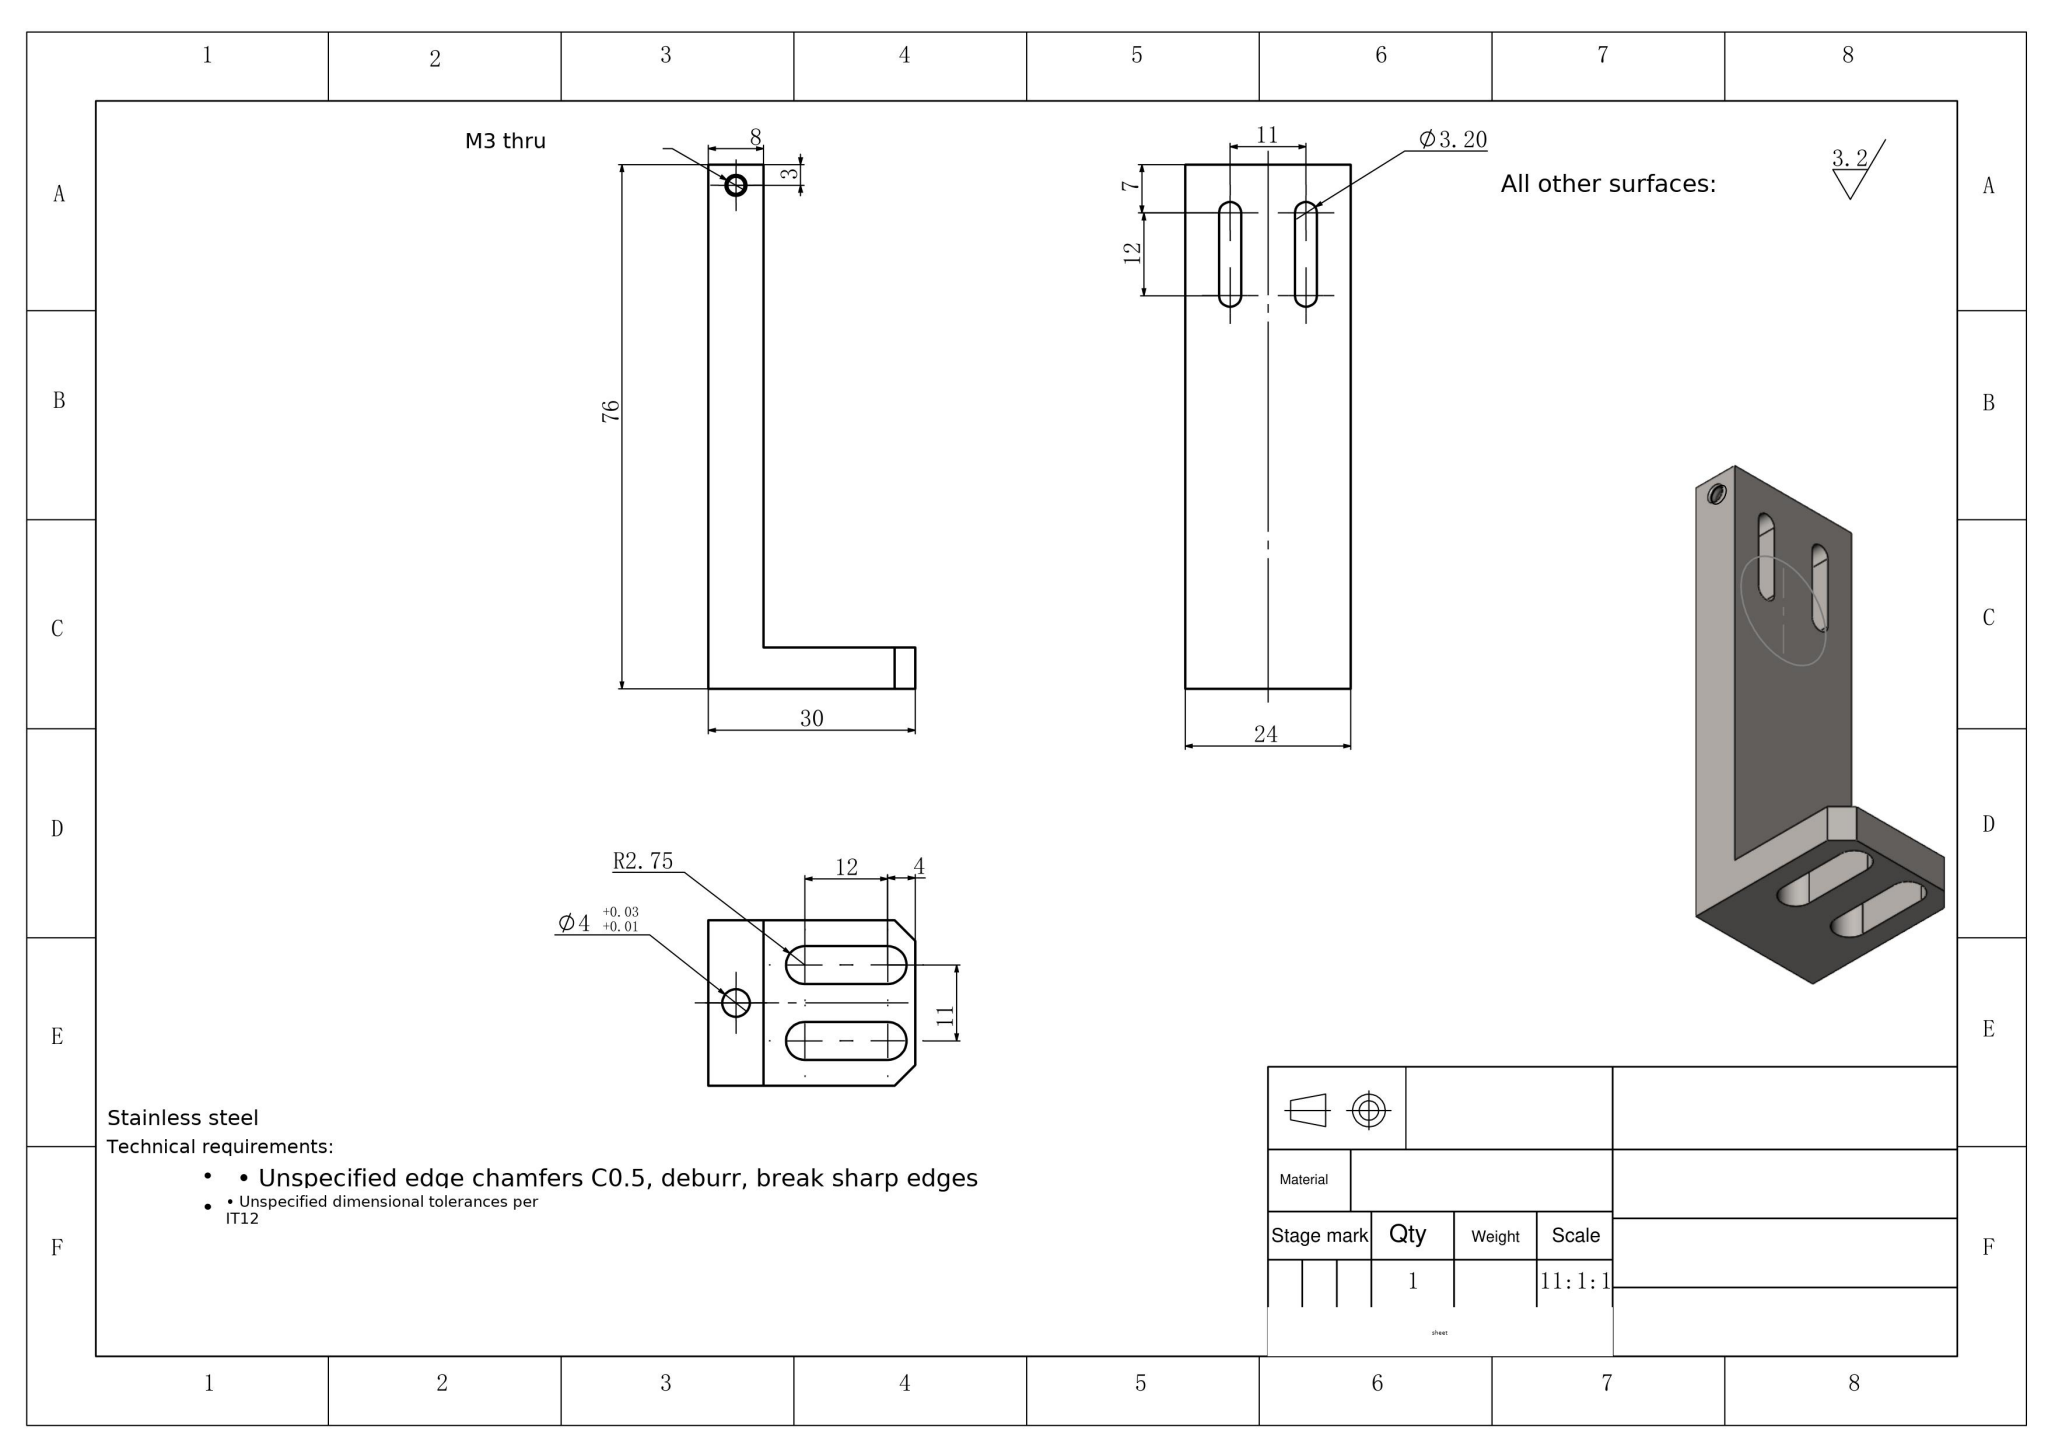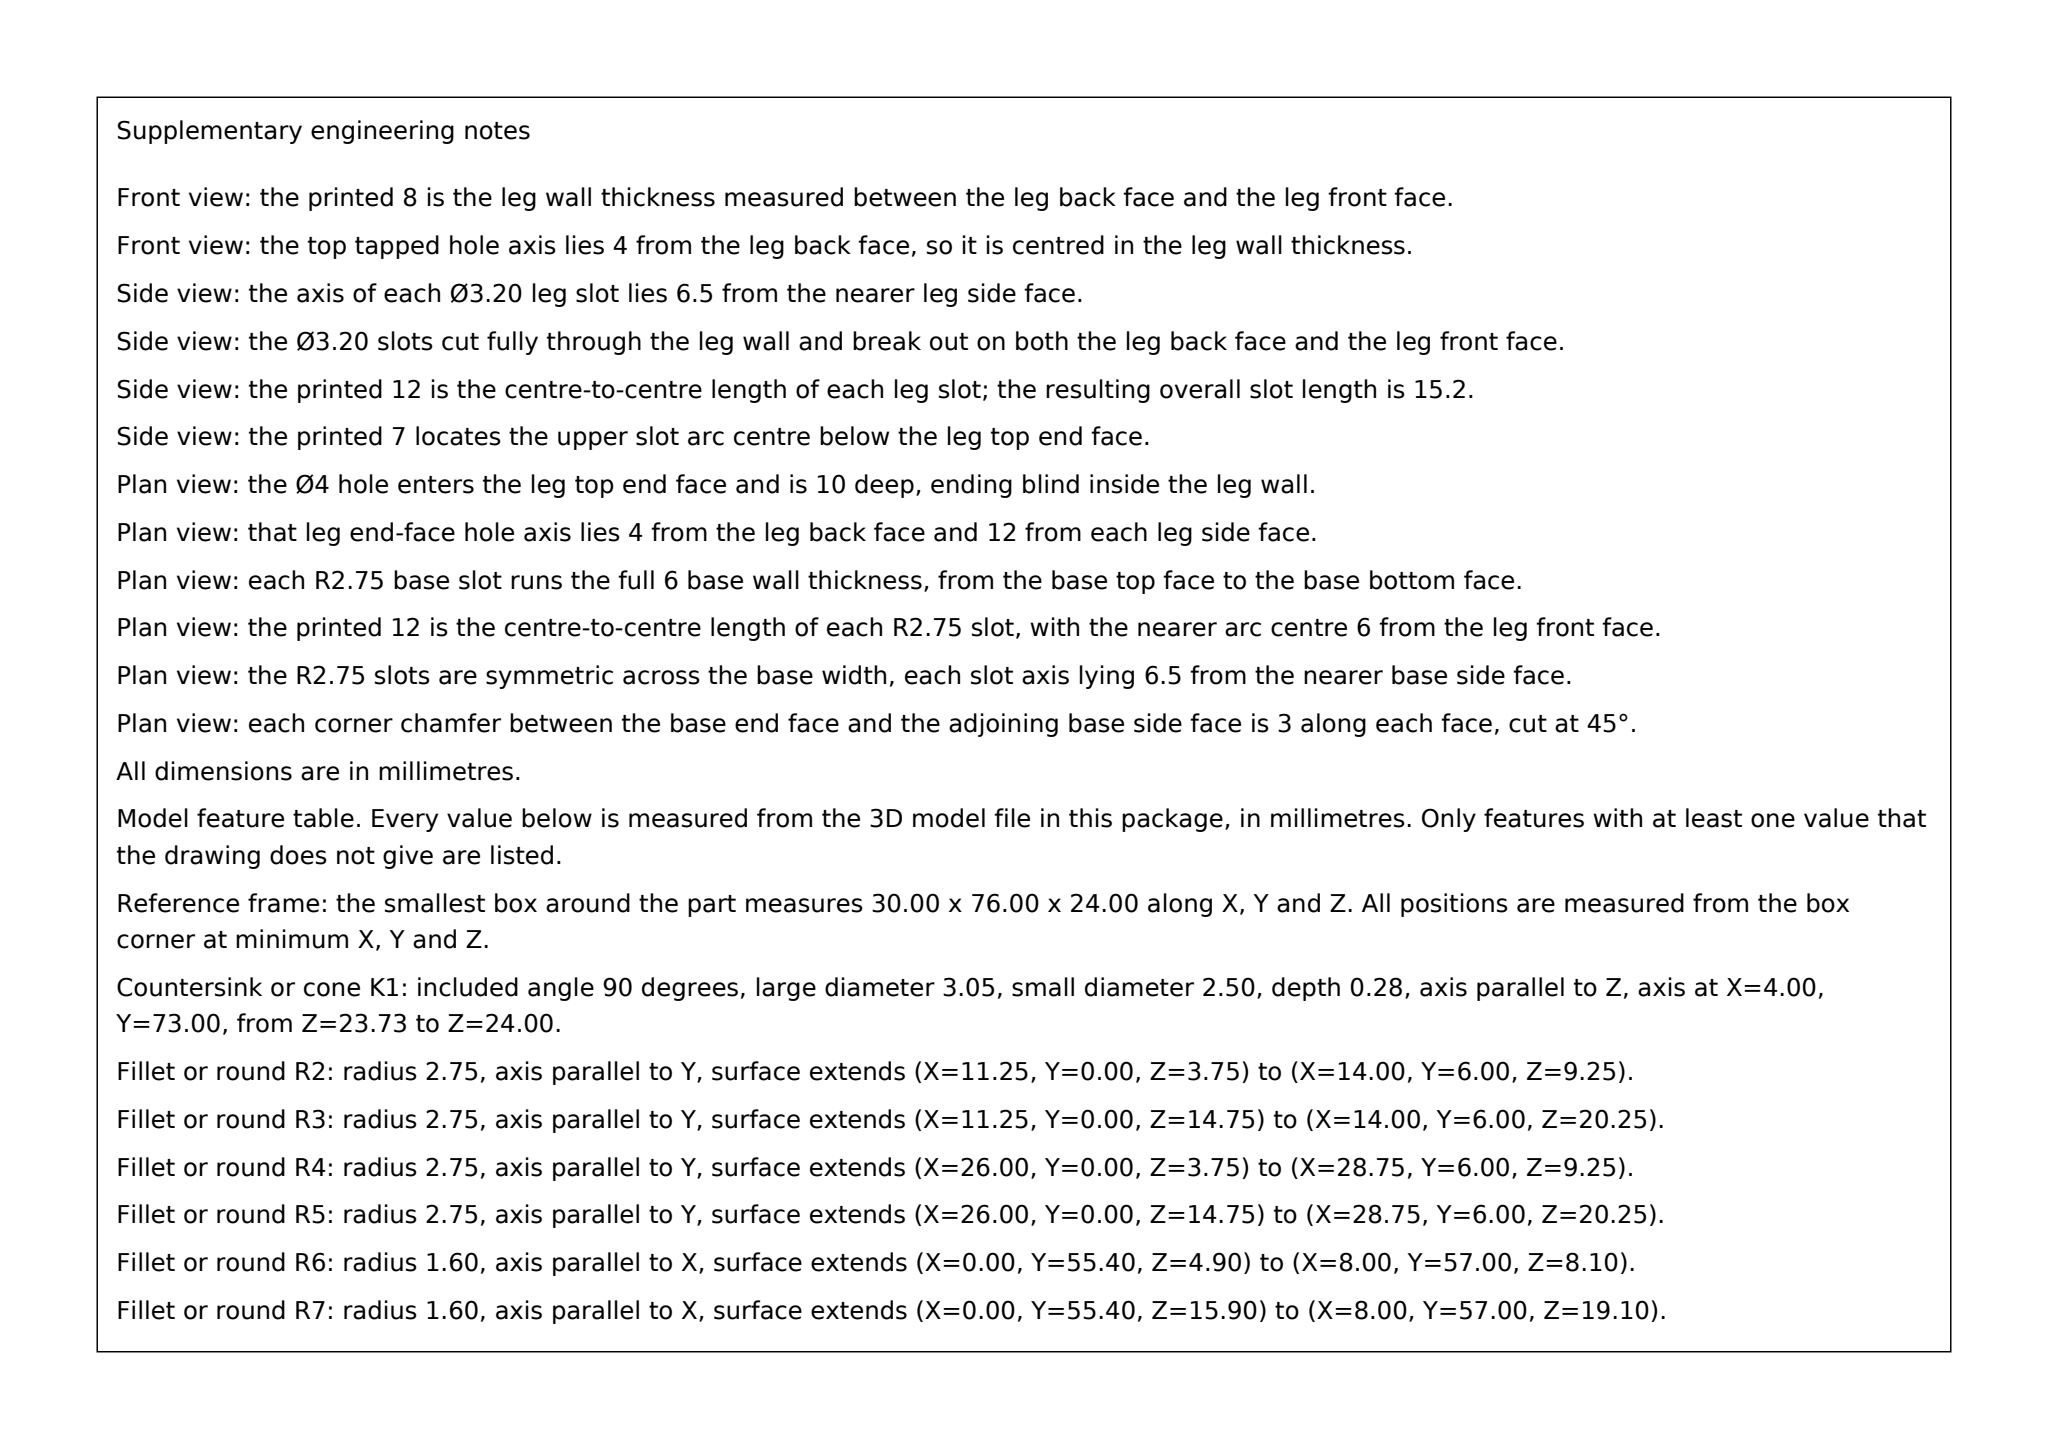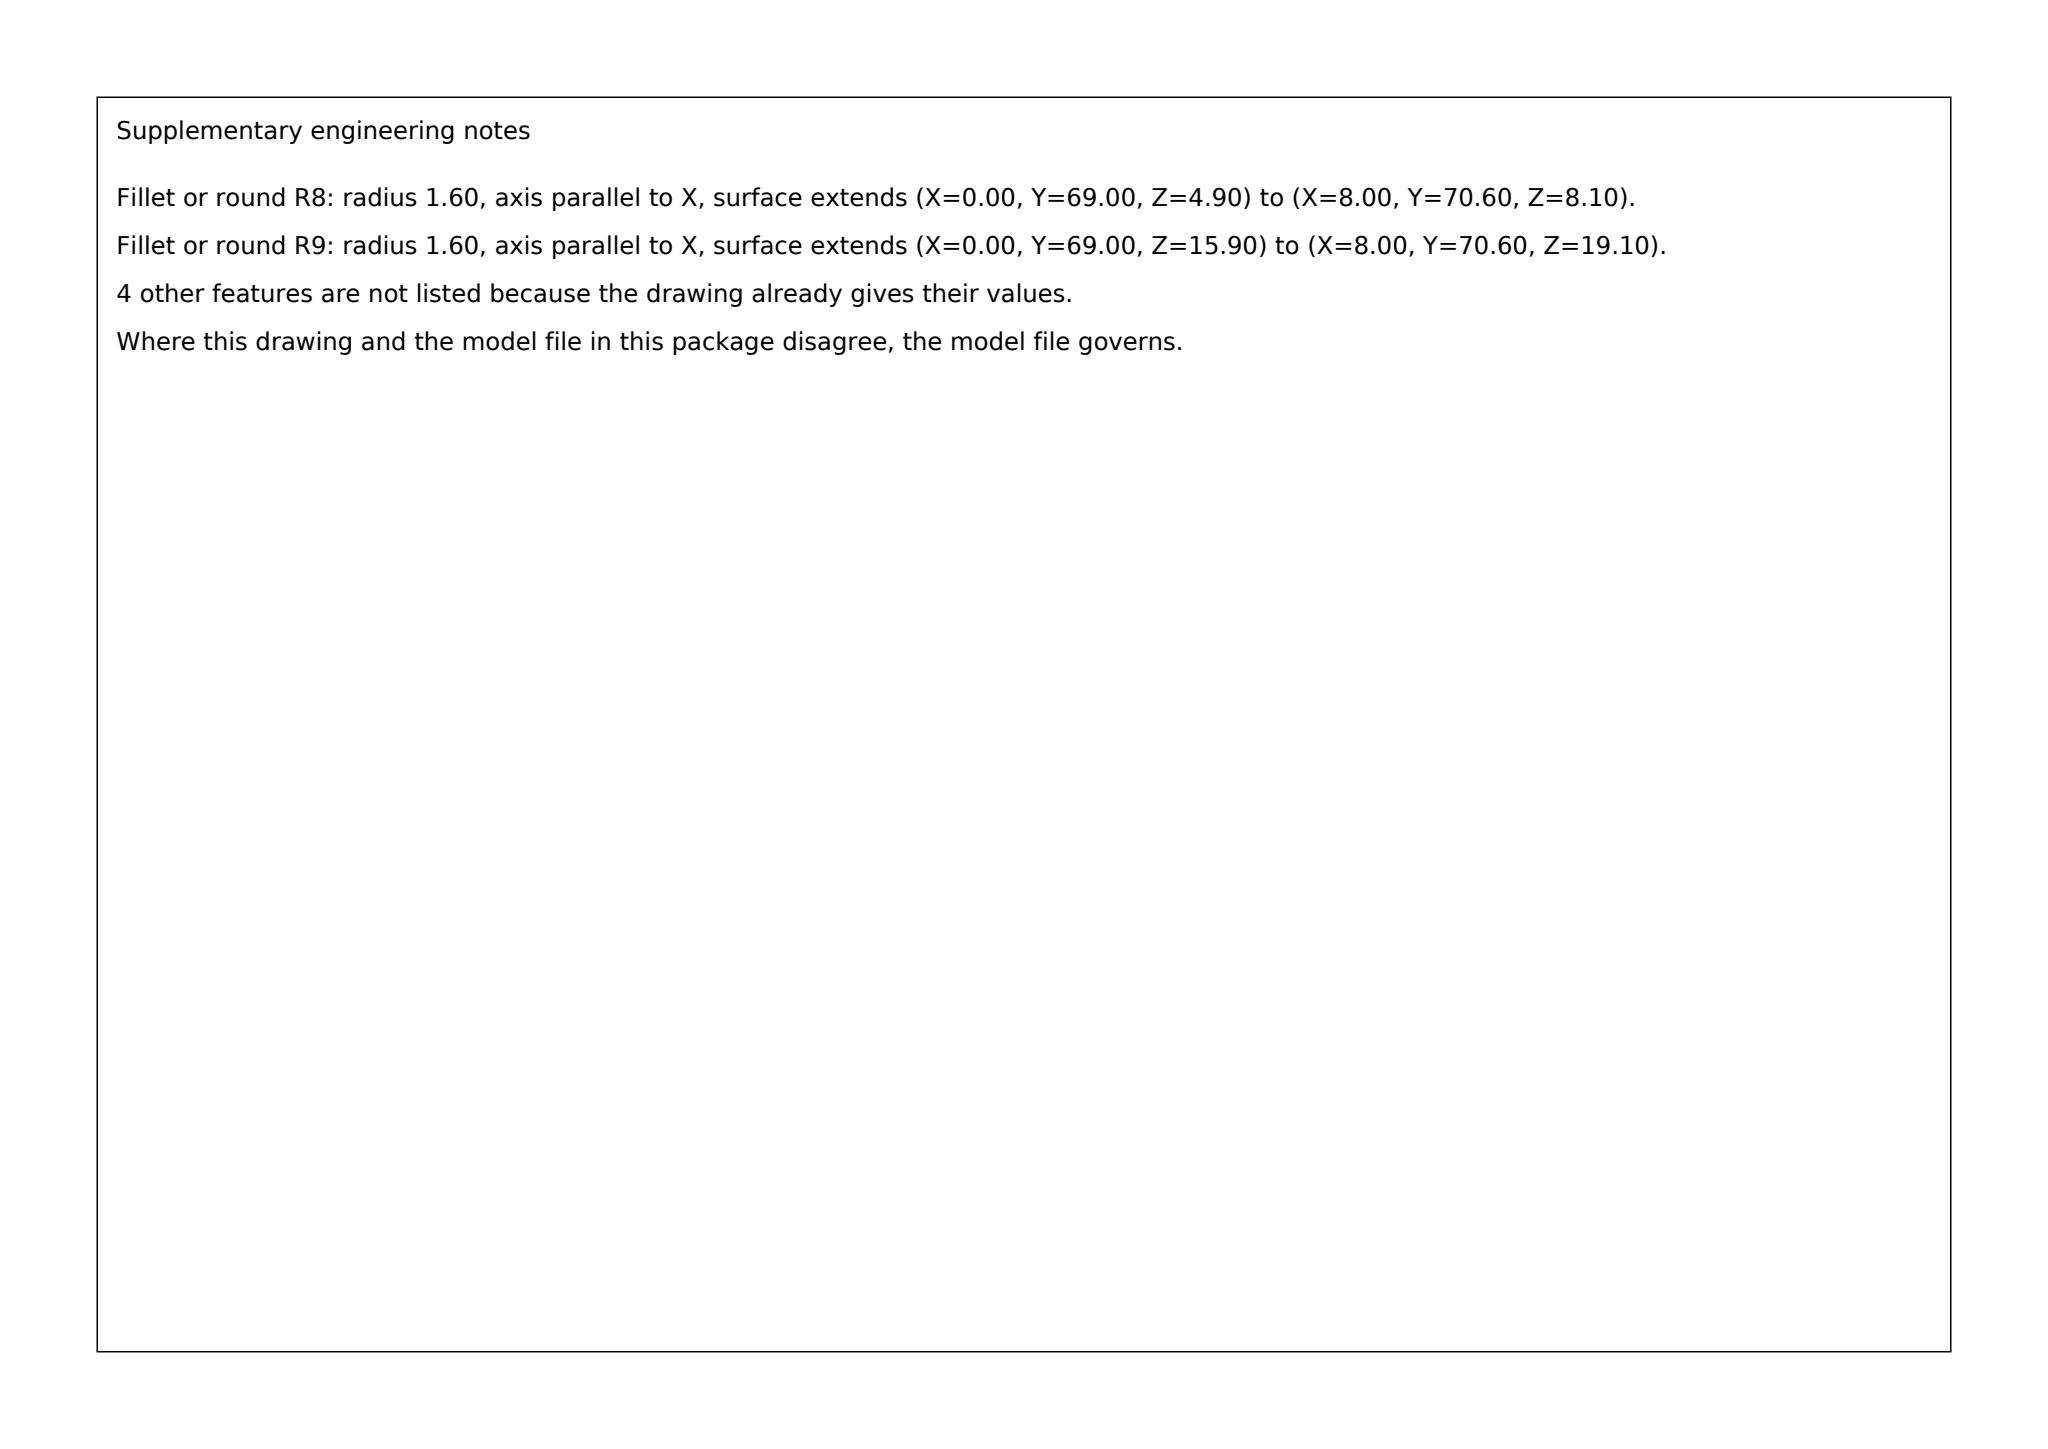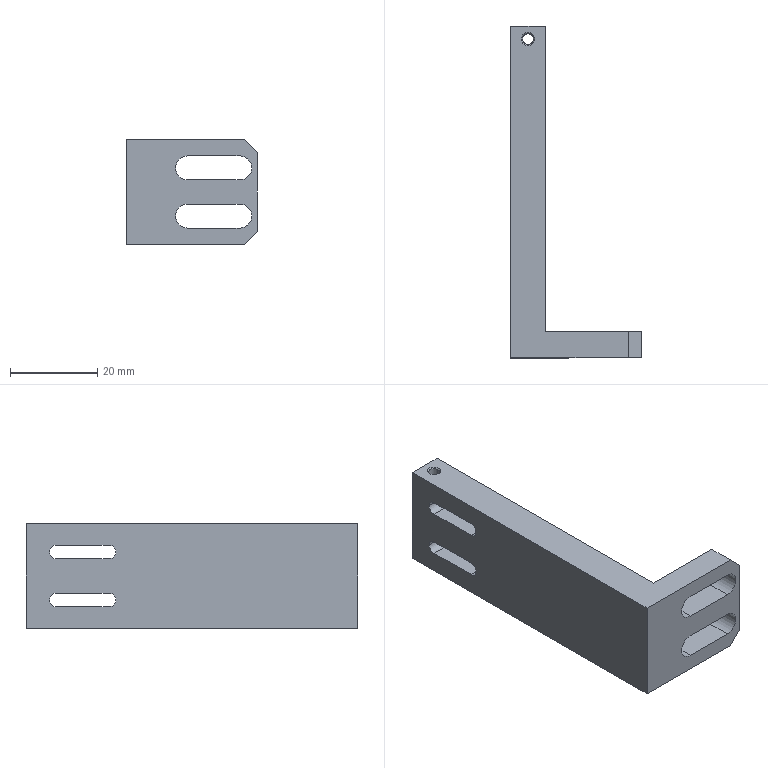Part | SolidWorks | mm | 1 solid | 39 faces | box 30 x 76 x 24 mm | volume 15661 mm3 | plane 19 | cylinder 18 | cone 2 | commonest cylinder face diameters 5.5 x6 3.2 x6 2.5 x4 4 x2
Drawing notes:
Ø4 +0.03/+0.01 hole in base: 10 deep (no counterbore), axis normal to base, located 4 from back face and 12 from either side face (centred in 24 width). | from the solid: cylinders[dia,axis,pos_other_axes,length]: [4.0,"y",[4.0,null,12.0],10.0]
M3 THRU: hole axis 4 from back face, i.e. centred in the 8 thick upright wall, and 3 from top face. | from the solid: cylinders[dia,axis,pos_other_axes,length]: [2.5,"z",[4.0,73.0,null],10.16/10.44] with planes x=0 and x=8
Base plate thickness 6 (from bottom face datum y=0 to underside of upright flange). | from the solid: axis_planes[normal_axis,offset]: y 0.0 and y 6.0
build123d program:
from build123d import *

# Parameters (mm, degrees)
BOSS_EXTRUDE1_DEPTH         = 24
CUT_EXTRUDE1_DEPTH          = 78.201
M3_TAPPED_HOLE1_D           = 2.5
M3_TAPPED_HOLE1_CSINK_D     = 3.05
M3_TAPPED_HOLE1_CSINK_ANGLE = 90
SKETCH5_R                   = 2
CUT_EXTRUDE2_DEPTH          = 10
CUT_EXTRUDE3_DEPTH          = 78.201
CHAMFER1_SIZE               = 3


with BuildPart() as part:
    # Sketch1 → Boss-Extrude1 (new body)
    with BuildSketch(Plane.XY):
        Polygon((0, 0), (0, 70), (-8, 70), (-8, -6), (22, -6), (22, 0), align=None)
    extrude(amount=BOSS_EXTRUDE1_DEPTH)

    # Sketch2 → Cut-Extrude1 (cut, through all)
    with BuildSketch(Plane(origin=(0, 0, 0), x_dir=(0, 0, -1), z_dir=(1, 0, 0))):
        with BuildLine():
            Line((-15.9, 63), (-15.9, 51))
            ThreePointArc((-15.9, 51), (-17.5, 49.4), (-19.1, 51))
            Line((-19.1, 51), (-19.1, 63))
            ThreePointArc((-19.1, 63), (-17.5, 64.6), (-15.9, 63))
        make_face()
        with BuildLine():
            Line((-4.9, 63), (-4.9, 51))
            ThreePointArc((-4.9, 51), (-6.5, 49.4), (-8.1, 51))
            Line((-8.1, 51), (-8.1, 63))
            ThreePointArc((-8.1, 63), (-6.5, 64.6), (-4.9, 63))
        make_face()
    extrude(amount=-CUT_EXTRUDE1_DEPTH, mode=Mode.SUBTRACT)

    # M3 Tapped Hole1 (through all)
    with Locations(Plane.XY.offset(24)):
        with Locations((-4, 67)):
            CounterSinkHole(M3_TAPPED_HOLE1_D / 2, M3_TAPPED_HOLE1_CSINK_D / 2, counter_sink_angle=M3_TAPPED_HOLE1_CSINK_ANGLE)

    # Sketch5 → Cut-Extrude2 (cut)
    with BuildSketch(Plane(origin=(0, 70, 0), x_dir=(1, 0, 0), z_dir=(0, 1, 0))):
        with Locations(Location((-4, -12, 0), (0, 0, 270))):
            Circle(SKETCH5_R)
    extrude(amount=-CUT_EXTRUDE2_DEPTH, mode=Mode.SUBTRACT)

    # Sketch6 → Cut-Extrude3 (cut, through all)
    with BuildSketch(Plane(origin=(0, 0, 0), x_dir=(1, 0, 0), z_dir=(0, 1, 0))):
        with BuildLine():
            Line((6, -14.75), (18, -14.75))
            ThreePointArc((18, -14.75), (20.75, -17.5), (18, -20.25))
            Line((18, -20.25), (6, -20.25))
            ThreePointArc((6, -20.25), (3.25, -17.5), (6, -14.75))
        make_face()
        with BuildLine():
            Line((6, -9.25), (18, -9.25))
            ThreePointArc((18, -9.25), (20.75, -6.5), (18, -3.75))
            Line((18, -3.75), (6, -3.75))
            ThreePointArc((6, -3.75), (3.25, -6.5), (6, -9.25))
        make_face()
    extrude(amount=-CUT_EXTRUDE3_DEPTH, mode=Mode.SUBTRACT)

    # Chamfer1
    chamfer1_edges = [part.edges().sort_by_distance(p)[0] for p in [
        (22, -3, 24),
        (22, -3, 0),
    ]]
    chamfer(chamfer1_edges, length=CHAMFER1_SIZE)


solid = part.part